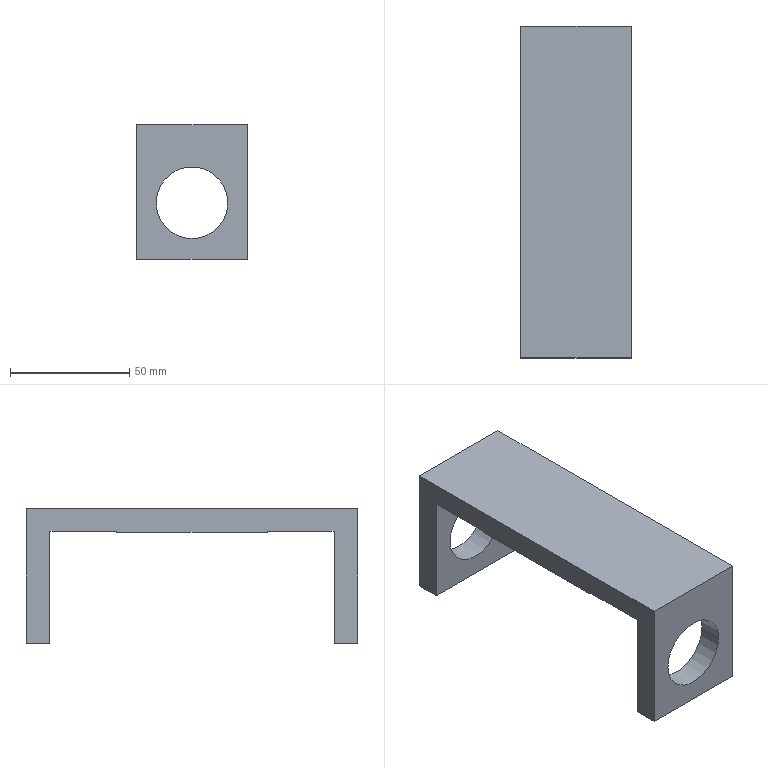Component | SolidWorks | HZ022-A001-D005-1 | 1 solid | 18 faces | box 46.5 x 139 x 56.5 mm | volume 92394 mm3 | plane 14 | cylinder 4 | commonest cylinder face diameters 30.05 x4 | material AL6061
build123d program:
from build123d import *

# Parameters (mm, degrees)
SKETCH1_2_W               = 139
SKETCH1_2_H               = 46.5
BOSS_EXTRUDE1_DEPTH       = 10
SKETCH2_W                 = 10
SKETCH2_H                 = 46.5
BOSS_EXTRUDE2_DEPTH       = 46.5
SKETCH3_R                 = 15.025
CUT_EXTRUDE1_DEPTH        = 152.835
SKETCH1_W                 = 28
SKETCH1_H                 = 60
CYLINDERCOVERRELIEF_DEPTH = 0.5


with BuildPart() as part:
    # Sketch1_2 → Boss-Extrude1 (new body)
    with BuildSketch(Plane(origin=(0, 0, 0), x_dir=(1, 0, 0), z_dir=(0, 1, 0))):
        Rectangle(SKETCH1_2_W, SKETCH1_2_H)
    extrude(amount=BOSS_EXTRUDE1_DEPTH)

    # Sketch2 → Boss-Extrude2 (add)
    with BuildSketch(Plane(origin=(0, 10, 0), x_dir=(1, 0, 0), z_dir=(0, 1, 0))):
        with Locations((-64.5, 0)):
            Rectangle(SKETCH2_W, SKETCH2_H)
        with Locations((64.5, 0)):
            Rectangle(SKETCH2_W, SKETCH2_H)
    extrude(amount=BOSS_EXTRUDE2_DEPTH)

    # Sketch3 → Cut-Extrude1 (cut, through all)
    with BuildSketch(Plane(origin=(69.5, 0, 0), x_dir=(0, 0, -1), z_dir=(1, 0, 0))):
        with Locations((0, 32.75)):
            Circle(SKETCH3_R)
    extrude(amount=-CUT_EXTRUDE1_DEPTH, mode=Mode.SUBTRACT)

    # Sketch1 → CylinderCoverRelief (cut)
    with BuildSketch(Plane(origin=(0, 10, 0), x_dir=(1, 0, 0), z_dir=(0, 1, 0))):
        with Locations((45.5, 0)):
            Rectangle(SKETCH1_W, SKETCH1_H)
        with Locations((-45.5, 0)):
            Rectangle(SKETCH1_W, SKETCH1_H)
    extrude(amount=-CYLINDERCOVERRELIEF_DEPTH, mode=Mode.SUBTRACT)


solid = part.part

# Placed as in the assembly
solid = solid.moved(Location((-12.865, -82.102, 400), (-90, 90, 0)))
STEP:
#1=COLOUR_RGB('',0.7922,0.8196,0.9333);
#2=FILL_AREA_STYLE_COLOUR('',#1);
#3=FILL_AREA_STYLE('',(#2));
#4=SURFACE_STYLE_FILL_AREA(#3);
#5=SURFACE_SIDE_STYLE('',(#4));
#6=SURFACE_STYLE_USAGE(.BOTH.,#5);
#7=PRESENTATION_STYLE_ASSIGNMENT((#6));
#8=CARTESIAN_POINT('',(0.08504,-0.4962,14.459));
#9=VERTEX_POINT('',#8);
#10=CARTESIAN_POINT('',(-1.098,-0.4962,14.459));
#11=VERTEX_POINT('',#10);
#12=CARTESIAN_POINT('',(-0.5065,-0.4962,14.459));
#13=DIRECTION('',(0.,-1.,0.));
#14=DIRECTION('',(-1.,0.,0.));
#15=AXIS2_PLACEMENT_3D('',#12,#13,#14);
#16=CIRCLE('',#15,0.5915);
#17=EDGE_CURVE('',#9,#11,#16,.T.);
#18=ORIENTED_EDGE('',*,*,#17,.F.);
#19=CARTESIAN_POINT('',(0.08504,-0.8899,14.459));
#20=VERTEX_POINT('',#19);
#21=CARTESIAN_POINT('',(0.08504,-0.4962,14.459));
#22=DIRECTION('',(0.,-1.,0.));
#23=VECTOR('',#22,39.37);
#24=LINE('',#21,#23);
#25=EDGE_CURVE('',#9,#20,#24,.T.);
#26=ORIENTED_EDGE('',*,*,#25,.T.);
#27=CARTESIAN_POINT('',(-1.098,-0.8899,14.459));
#28=VERTEX_POINT('',#27);
#29=CARTESIAN_POINT('',(-0.5065,-0.8899,14.459));
#30=DIRECTION('',(-0.,1.,-0.));
#31=DIRECTION('',(1.,0.,0.));
#32=AXIS2_PLACEMENT_3D('',#29,#30,#31);
#33=CIRCLE('',#32,0.5915);
#34=EDGE_CURVE('',#28,#20,#33,.T.);
#35=ORIENTED_EDGE('',*,*,#34,.F.);
#36=CARTESIAN_POINT('',(-1.098,-0.4962,14.459));
#37=DIRECTION('',(0.,-1.,0.));
#38=VECTOR('',#37,39.37);
#39=LINE('',#36,#38);
#40=EDGE_CURVE('',#11,#28,#39,.T.);
#41=ORIENTED_EDGE('',*,*,#40,.F.);
#42=EDGE_LOOP('',(#18,#26,#35,#41));
#43=FACE_OUTER_BOUND('',#42,.T.);
#44=CARTESIAN_POINT('',(-0.5065,-0.4962,14.459));
#45=DIRECTION('',(0.,-1.,0.));
#46=DIRECTION('',(-1.,0.,0.));
#47=AXIS2_PLACEMENT_3D('',#44,#45,#46);
#48=CYLINDRICAL_SURFACE('',#47,0.5915);
#49=ADVANCED_FACE('',(#43),#48,.F.);
#50=CARTESIAN_POINT('',(0.08504,-5.575,14.459));
#51=VERTEX_POINT('',#50);
#52=CARTESIAN_POINT('',(-1.098,-5.575,14.459));
#53=VERTEX_POINT('',#52);
#54=CARTESIAN_POINT('',(-0.5065,-5.575,14.459));
#55=DIRECTION('',(-0.,-1.,-0.));
#56=DIRECTION('',(-1.,0.,0.));
#57=AXIS2_PLACEMENT_3D('',#54,#55,#56);
#58=CIRCLE('',#57,0.5915);
#59=EDGE_CURVE('',#51,#53,#58,.T.);
#60=ORIENTED_EDGE('',*,*,#59,.F.);
#61=CARTESIAN_POINT('',(0.08504,-5.969,14.459));
#62=VERTEX_POINT('',#61);
#63=CARTESIAN_POINT('',(0.08504,-0.4962,14.459));
#64=DIRECTION('',(0.,-1.,0.));
#65=VECTOR('',#64,39.37);
#66=LINE('',#63,#65);
#67=EDGE_CURVE('',#51,#62,#66,.T.);
#68=ORIENTED_EDGE('',*,*,#67,.T.);
#69=CARTESIAN_POINT('',(-1.098,-5.969,14.459));
#70=VERTEX_POINT('',#69);
#71=CARTESIAN_POINT('',(-0.5065,-5.969,14.459));
#72=DIRECTION('',(0.,-1.,0.));
#73=DIRECTION('',(-1.,0.,0.));
#74=AXIS2_PLACEMENT_3D('',#71,#72,#73);
#75=CIRCLE('',#74,0.5915);
#76=EDGE_CURVE('',#62,#70,#75,.T.);
#77=ORIENTED_EDGE('',*,*,#76,.T.);
#78=CARTESIAN_POINT('',(-1.098,-0.4962,14.459));
#79=DIRECTION('',(0.,-1.,0.));
#80=VECTOR('',#79,39.37);
#81=LINE('',#78,#80);
#82=EDGE_CURVE('',#53,#70,#81,.T.);
#83=ORIENTED_EDGE('',*,*,#82,.F.);
#84=EDGE_LOOP('',(#60,#68,#77,#83));
#85=FACE_OUTER_BOUND('',#84,.T.);
#86=CARTESIAN_POINT('',(-0.5065,-0.4962,14.459));
#87=DIRECTION('',(0.,-1.,0.));
#88=DIRECTION('',(-1.,0.,0.));
#89=AXIS2_PLACEMENT_3D('',#86,#87,#88);
#90=CYLINDRICAL_SURFACE('',#89,0.5915);
#91=ADVANCED_FACE('',(#85),#90,.F.);
#92=CARTESIAN_POINT('',(-1.422,-4.473,15.354));
#93=VERTEX_POINT('',#92);
#94=CARTESIAN_POINT('',(0.4089,-4.473,15.354));
#95=VERTEX_POINT('',#94);
#96=CARTESIAN_POINT('',(0.6746,-4.473,15.354));
#97=DIRECTION('',(1.,-0.,0.));
#98=VECTOR('',#97,39.37);
#99=LINE('',#96,#98);
#100=EDGE_CURVE('',#93,#95,#99,.T.);
#101=ORIENTED_EDGE('',*,*,#100,.F.);
#102=CARTESIAN_POINT('',(-1.422,-1.992,15.354));
#103=VERTEX_POINT('',#102);
#104=CARTESIAN_POINT('',(-1.422,-0.4962,15.354));
#105=DIRECTION('',(-0.,1.,-0.));
#106=VECTOR('',#105,39.37);
#107=LINE('',#104,#106);
#108=EDGE_CURVE('',#93,#103,#107,.T.);
#109=ORIENTED_EDGE('',*,*,#108,.T.);
#110=CARTESIAN_POINT('',(0.4089,-1.992,15.354));
#111=VERTEX_POINT('',#110);
#112=CARTESIAN_POINT('',(-1.688,-1.992,15.354));
#113=DIRECTION('',(-1.,0.,-0.));
#114=VECTOR('',#113,39.37);
#115=LINE('',#112,#114);
#116=EDGE_CURVE('',#111,#103,#115,.T.);
#117=ORIENTED_EDGE('',*,*,#116,.F.);
#118=CARTESIAN_POINT('',(0.4089,-0.4962,15.354));
#119=DIRECTION('',(0.,-1.,0.));
#120=VECTOR('',#119,39.37);
#121=LINE('',#118,#120);
#122=EDGE_CURVE('',#111,#95,#121,.T.);
#123=ORIENTED_EDGE('',*,*,#122,.T.);
#124=EDGE_LOOP('',(#101,#109,#117,#123));
#125=FACE_OUTER_BOUND('',#124,.T.);
#126=CARTESIAN_POINT('',(-0.5065,-3.232,15.354));
#127=DIRECTION('',(0.,0.,-1.));
#128=DIRECTION('',(1.,-0.,0.));
#129=AXIS2_PLACEMENT_3D('',#126,#127,#128);
#130=PLANE('',#129);
#131=ADVANCED_FACE('',(#125),#130,.T.);
#132=CARTESIAN_POINT('',(-0.5065,-5.969,14.459));
#133=DIRECTION('',(0.,-1.,0.));
#134=DIRECTION('',(-1.,0.,0.));
#135=AXIS2_PLACEMENT_3D('',#132,#133,#134);
#136=CIRCLE('',#135,0.5915);
#137=EDGE_CURVE('',#70,#62,#136,.T.);
#138=ORIENTED_EDGE('',*,*,#137,.F.);
#139=ORIENTED_EDGE('',*,*,#76,.F.);
#140=EDGE_LOOP('',(#138,#139));
#141=FACE_BOUND('',#140,.T.);
#142=CARTESIAN_POINT('',(0.4089,-5.969,15.748));
#143=VERTEX_POINT('',#142);
#144=CARTESIAN_POINT('',(-1.422,-5.969,15.748));
#145=VERTEX_POINT('',#144);
#146=CARTESIAN_POINT('',(-1.422,-5.969,15.748));
#147=DIRECTION('',(-1.,0.,-0.));
#148=VECTOR('',#147,39.37);
#149=LINE('',#146,#148);
#150=EDGE_CURVE('',#143,#145,#149,.T.);
#151=ORIENTED_EDGE('',*,*,#150,.T.);
#152=CARTESIAN_POINT('',(-1.422,-5.969,13.524));
#153=VERTEX_POINT('',#152);
#154=CARTESIAN_POINT('',(-1.422,-5.969,15.354));
#155=DIRECTION('',(-0.,-0.,1.));
#156=VECTOR('',#155,39.37);
#157=LINE('',#154,#156);
#158=EDGE_CURVE('',#153,#145,#157,.T.);
#159=ORIENTED_EDGE('',*,*,#158,.F.);
#160=CARTESIAN_POINT('',(0.4089,-5.969,13.524));
#161=VERTEX_POINT('',#160);
#162=CARTESIAN_POINT('',(0.4089,-5.969,13.524));
#163=DIRECTION('',(-1.,0.,-0.));
#164=VECTOR('',#163,39.37);
#165=LINE('',#162,#164);
#166=EDGE_CURVE('',#161,#153,#165,.T.);
#167=ORIENTED_EDGE('',*,*,#166,.F.);
#168=CARTESIAN_POINT('',(0.4089,-5.969,15.354));
#169=DIRECTION('',(-0.,-0.,1.));
#170=VECTOR('',#169,39.37);
#171=LINE('',#168,#170);
#172=EDGE_CURVE('',#161,#143,#171,.T.);
#173=ORIENTED_EDGE('',*,*,#172,.T.);
#174=EDGE_LOOP('',(#151,#159,#167,#173));
#175=FACE_OUTER_BOUND('',#174,.T.);
#176=CARTESIAN_POINT('',(-1.422,-5.969,15.354));
#177=DIRECTION('',(0.,1.,-0.));
#178=DIRECTION('',(1.,-0.,0.));
#179=AXIS2_PLACEMENT_3D('',#176,#177,#178);
#180=PLANE('',#179);
#181=ADVANCED_FACE('',(#141,#175),#180,.F.);
#182=ORIENTED_EDGE('',*,*,#108,.F.);
#183=CARTESIAN_POINT('',(-1.422,-4.473,15.374));
#184=VERTEX_POINT('',#183);
#185=CARTESIAN_POINT('',(-1.422,-4.473,15.354));
#186=DIRECTION('',(-0.,-0.,1.));
#187=VECTOR('',#186,39.37);
#188=LINE('',#185,#187);
#189=EDGE_CURVE('',#93,#184,#188,.T.);
#190=ORIENTED_EDGE('',*,*,#189,.T.);
#191=CARTESIAN_POINT('',(-1.422,-5.575,15.374));
#192=VERTEX_POINT('',#191);
#193=CARTESIAN_POINT('',(-1.422,-0.4962,15.374));
#194=DIRECTION('',(0.,-1.,0.));
#195=VECTOR('',#194,39.37);
#196=LINE('',#193,#195);
#197=EDGE_CURVE('',#184,#192,#196,.T.);
#198=ORIENTED_EDGE('',*,*,#197,.T.);
#199=CARTESIAN_POINT('',(-1.422,-5.575,13.524));
#200=VERTEX_POINT('',#199);
#201=CARTESIAN_POINT('',(-1.422,-5.575,13.524));
#202=DIRECTION('',(-0.,-0.,1.));
#203=VECTOR('',#202,39.37);
#204=LINE('',#201,#203);
#205=EDGE_CURVE('',#200,#192,#204,.T.);
#206=ORIENTED_EDGE('',*,*,#205,.F.);
#207=CARTESIAN_POINT('',(-1.422,-5.575,13.524));
#208=DIRECTION('',(-0.,1.,-0.));
#209=VECTOR('',#208,39.37);
#210=LINE('',#207,#209);
#211=EDGE_CURVE('',#153,#200,#210,.T.);
#212=ORIENTED_EDGE('',*,*,#211,.F.);
#213=ORIENTED_EDGE('',*,*,#158,.T.);
#214=CARTESIAN_POINT('',(-1.422,-0.4962,15.748));
#215=VERTEX_POINT('',#214);
#216=CARTESIAN_POINT('',(-1.422,-0.4962,15.748));
#217=DIRECTION('',(-0.,1.,-0.));
#218=VECTOR('',#217,39.37);
#219=LINE('',#216,#218);
#220=EDGE_CURVE('',#145,#215,#219,.T.);
#221=ORIENTED_EDGE('',*,*,#220,.T.);
#222=CARTESIAN_POINT('',(-1.422,-0.4962,13.524));
#223=VERTEX_POINT('',#222);
#224=CARTESIAN_POINT('',(-1.422,-0.4962,15.354));
#225=DIRECTION('',(-0.,-0.,1.));
#226=VECTOR('',#225,39.37);
#227=LINE('',#224,#226);
#228=EDGE_CURVE('',#223,#215,#227,.T.);
#229=ORIENTED_EDGE('',*,*,#228,.F.);
#230=CARTESIAN_POINT('',(-1.422,-0.8899,13.524));
#231=VERTEX_POINT('',#230);
#232=CARTESIAN_POINT('',(-1.422,-0.8899,13.524));
#233=DIRECTION('',(-0.,1.,-0.));
#234=VECTOR('',#233,39.37);
#235=LINE('',#232,#234);
#236=EDGE_CURVE('',#231,#223,#235,.T.);
#237=ORIENTED_EDGE('',*,*,#236,.F.);
#238=CARTESIAN_POINT('',(-1.422,-0.8899,15.374));
#239=VERTEX_POINT('',#238);
#240=CARTESIAN_POINT('',(-1.422,-0.8899,13.524));
#241=DIRECTION('',(-0.,-0.,1.));
#242=VECTOR('',#241,39.37);
#243=LINE('',#240,#242);
#244=EDGE_CURVE('',#231,#239,#243,.T.);
#245=ORIENTED_EDGE('',*,*,#244,.T.);
#246=CARTESIAN_POINT('',(-1.422,-1.992,15.374));
#247=VERTEX_POINT('',#246);
#248=CARTESIAN_POINT('',(-1.422,-0.4962,15.374));
#249=DIRECTION('',(0.,-1.,0.));
#250=VECTOR('',#249,39.37);
#251=LINE('',#248,#250);
#252=EDGE_CURVE('',#239,#247,#251,.T.);
#253=ORIENTED_EDGE('',*,*,#252,.T.);
#254=CARTESIAN_POINT('',(-1.422,-1.992,15.354));
#255=DIRECTION('',(0.,0.,-1.));
#256=VECTOR('',#255,39.37);
#257=LINE('',#254,#256);
#258=EDGE_CURVE('',#247,#103,#257,.T.);
#259=ORIENTED_EDGE('',*,*,#258,.T.);
#260=EDGE_LOOP('',(#182,#190,#198,#206,#212,#213,#221,#229,#237,#245,#253,#259));
#261=FACE_OUTER_BOUND('',#260,.T.);
#262=CARTESIAN_POINT('',(-1.422,-0.4962,15.354));
#263=DIRECTION('',(1.,0.,0.));
#264=DIRECTION('',(0.,-1.,0.));
#265=AXIS2_PLACEMENT_3D('',#262,#263,#264);
#266=PLANE('',#265);
#267=ADVANCED_FACE('',(#261),#266,.F.);
#268=CARTESIAN_POINT('',(-0.5065,-0.4962,14.459));
#269=DIRECTION('',(0.,-1.,0.));
#270=DIRECTION('',(-1.,0.,0.));
#271=AXIS2_PLACEMENT_3D('',#268,#269,#270);
#272=CIRCLE('',#271,0.5915);
#273=EDGE_CURVE('',#11,#9,#272,.T.);
#274=ORIENTED_EDGE('',*,*,#273,.T.);
#275=ORIENTED_EDGE('',*,*,#17,.T.);
#276=EDGE_LOOP('',(#274,#275));
#277=FACE_BOUND('',#276,.T.);
#278=CARTESIAN_POINT('',(0.4089,-0.4962,15.748));
#279=VERTEX_POINT('',#278);
#280=CARTESIAN_POINT('',(-1.422,-0.4962,15.748));
#281=DIRECTION('',(1.,-0.,0.));
#282=VECTOR('',#281,39.37);
#283=LINE('',#280,#282);
#284=EDGE_CURVE('',#215,#279,#283,.T.);
#285=ORIENTED_EDGE('',*,*,#284,.T.);
#286=CARTESIAN_POINT('',(0.4089,-0.4962,13.524));
#287=VERTEX_POINT('',#286);
#288=CARTESIAN_POINT('',(0.4089,-0.4962,15.354));
#289=DIRECTION('',(-0.,-0.,1.));
#290=VECTOR('',#289,39.37);
#291=LINE('',#288,#290);
#292=EDGE_CURVE('',#287,#279,#291,.T.);
#293=ORIENTED_EDGE('',*,*,#292,.F.);
#294=CARTESIAN_POINT('',(0.4089,-0.4962,13.524));
#295=DIRECTION('',(1.,-0.,0.));
#296=VECTOR('',#295,39.37);
#297=LINE('',#294,#296);
#298=EDGE_CURVE('',#223,#287,#297,.T.);
#299=ORIENTED_EDGE('',*,*,#298,.F.);
#300=ORIENTED_EDGE('',*,*,#228,.T.);
#301=EDGE_LOOP('',(#285,#293,#299,#300));
#302=FACE_OUTER_BOUND('',#301,.T.);
#303=CARTESIAN_POINT('',(-1.422,-0.4962,15.354));
#304=DIRECTION('',(-0.,-1.,0.));
#305=DIRECTION('',(-1.,0.,-0.));
#306=AXIS2_PLACEMENT_3D('',#303,#304,#305);
#307=PLANE('',#306);
#308=ADVANCED_FACE('',(#277,#302),#307,.F.);
#309=CARTESIAN_POINT('',(0.4089,-5.575,15.374));
#310=VERTEX_POINT('',#309);
#311=CARTESIAN_POINT('',(0.4089,-4.473,15.374));
#312=VERTEX_POINT('',#311);
#313=CARTESIAN_POINT('',(0.4089,-0.4962,15.374));
#314=DIRECTION('',(-0.,1.,-0.));
#315=VECTOR('',#314,39.37);
#316=LINE('',#313,#315);
#317=EDGE_CURVE('',#310,#312,#316,.T.);
#318=ORIENTED_EDGE('',*,*,#317,.T.);
#319=CARTESIAN_POINT('',(0.4089,-4.473,15.354));
#320=DIRECTION('',(0.,0.,-1.));
#321=VECTOR('',#320,39.37);
#322=LINE('',#319,#321);
#323=EDGE_CURVE('',#312,#95,#322,.T.);
#324=ORIENTED_EDGE('',*,*,#323,.T.);
#325=ORIENTED_EDGE('',*,*,#122,.F.);
#326=CARTESIAN_POINT('',(0.4089,-1.992,15.374));
#327=VERTEX_POINT('',#326);
#328=CARTESIAN_POINT('',(0.4089,-1.992,15.354));
#329=DIRECTION('',(-0.,-0.,1.));
#330=VECTOR('',#329,39.37);
#331=LINE('',#328,#330);
#332=EDGE_CURVE('',#111,#327,#331,.T.);
#333=ORIENTED_EDGE('',*,*,#332,.T.);
#334=CARTESIAN_POINT('',(0.4089,-0.8899,15.374));
#335=VERTEX_POINT('',#334);
#336=CARTESIAN_POINT('',(0.4089,-0.4962,15.374));
#337=DIRECTION('',(-0.,1.,-0.));
#338=VECTOR('',#337,39.37);
#339=LINE('',#336,#338);
#340=EDGE_CURVE('',#327,#335,#339,.T.);
#341=ORIENTED_EDGE('',*,*,#340,.T.);
#342=CARTESIAN_POINT('',(0.4089,-0.8899,13.524));
#343=VERTEX_POINT('',#342);
#344=CARTESIAN_POINT('',(0.4089,-0.8899,13.524));
#345=DIRECTION('',(-0.,-0.,1.));
#346=VECTOR('',#345,39.37);
#347=LINE('',#344,#346);
#348=EDGE_CURVE('',#343,#335,#347,.T.);
#349=ORIENTED_EDGE('',*,*,#348,.F.);
#350=CARTESIAN_POINT('',(0.4089,-0.8899,13.524));
#351=DIRECTION('',(0.,-1.,0.));
#352=VECTOR('',#351,39.37);
#353=LINE('',#350,#352);
#354=EDGE_CURVE('',#287,#343,#353,.T.);
#355=ORIENTED_EDGE('',*,*,#354,.F.);
#356=ORIENTED_EDGE('',*,*,#292,.T.);
#357=CARTESIAN_POINT('',(0.4089,-0.4962,15.748));
#358=DIRECTION('',(0.,-1.,0.));
#359=VECTOR('',#358,39.37);
#360=LINE('',#357,#359);
#361=EDGE_CURVE('',#279,#143,#360,.T.);
#362=ORIENTED_EDGE('',*,*,#361,.T.);
#363=ORIENTED_EDGE('',*,*,#172,.F.);
#364=CARTESIAN_POINT('',(0.4089,-5.575,13.524));
#365=VERTEX_POINT('',#364);
#366=CARTESIAN_POINT('',(0.4089,-5.575,13.524));
#367=DIRECTION('',(-0.,-1.,-0.));
#368=VECTOR('',#367,39.37);
#369=LINE('',#366,#368);
#370=EDGE_CURVE('',#365,#161,#369,.T.);
#371=ORIENTED_EDGE('',*,*,#370,.F.);
#372=CARTESIAN_POINT('',(0.4089,-5.575,13.524));
#373=DIRECTION('',(-0.,-0.,1.));
#374=VECTOR('',#373,39.37);
#375=LINE('',#372,#374);
#376=EDGE_CURVE('',#365,#310,#375,.T.);
#377=ORIENTED_EDGE('',*,*,#376,.T.);
#378=EDGE_LOOP('',(#318,#324,#325,#333,#341,#349,#355,#356,#362,#363,#371,#377));
#379=FACE_OUTER_BOUND('',#378,.T.);
#380=CARTESIAN_POINT('',(0.4089,-0.4962,15.354));
#381=DIRECTION('',(-1.,-0.,-0.));
#382=DIRECTION('',(-0.,1.,-0.));
#383=AXIS2_PLACEMENT_3D('',#380,#381,#382);
#384=PLANE('',#383);
#385=ADVANCED_FACE('',(#379),#384,.F.);
#386=ORIENTED_EDGE('',*,*,#150,.F.);
#387=ORIENTED_EDGE('',*,*,#361,.F.);
#388=ORIENTED_EDGE('',*,*,#284,.F.);
#389=ORIENTED_EDGE('',*,*,#220,.F.);
#390=EDGE_LOOP('',(#386,#387,#388,#389));
#391=FACE_OUTER_BOUND('',#390,.T.);
#392=CARTESIAN_POINT('',(-0.5065,-3.232,15.748));
#393=DIRECTION('',(0.,0.,-1.));
#394=DIRECTION('',(1.,-0.,0.));
#395=AXIS2_PLACEMENT_3D('',#392,#393,#394);
#396=PLANE('',#395);
#397=ADVANCED_FACE('',(#391),#396,.F.);
#398=ORIENTED_EDGE('',*,*,#34,.T.);
#399=CARTESIAN_POINT('',(-0.5065,-0.8899,14.459));
#400=DIRECTION('',(-0.,1.,-0.));
#401=DIRECTION('',(1.,0.,0.));
#402=AXIS2_PLACEMENT_3D('',#399,#400,#401);
#403=CIRCLE('',#402,0.5915);
#404=EDGE_CURVE('',#20,#28,#403,.T.);
#405=ORIENTED_EDGE('',*,*,#404,.T.);
#406=EDGE_LOOP('',(#398,#405));
#407=FACE_BOUND('',#406,.T.);
#408=ORIENTED_EDGE('',*,*,#348,.T.);
#409=CARTESIAN_POINT('',(0.6746,-0.8899,15.374));
#410=DIRECTION('',(1.,-0.,0.));
#411=VECTOR('',#410,39.37);
#412=LINE('',#409,#411);
#413=EDGE_CURVE('',#239,#335,#412,.T.);
#414=ORIENTED_EDGE('',*,*,#413,.F.);
#415=ORIENTED_EDGE('',*,*,#244,.F.);
#416=CARTESIAN_POINT('',(0.4089,-0.8899,13.524));
#417=DIRECTION('',(-1.,0.,-0.));
#418=VECTOR('',#417,39.37);
#419=LINE('',#416,#418);
#420=EDGE_CURVE('',#343,#231,#419,.T.);
#421=ORIENTED_EDGE('',*,*,#420,.F.);
#422=EDGE_LOOP('',(#408,#414,#415,#421));
#423=FACE_OUTER_BOUND('',#422,.T.);
#424=CARTESIAN_POINT('',(0.4089,-0.8899,13.524));
#425=DIRECTION('',(0.,1.,-0.));
#426=DIRECTION('',(1.,-0.,0.));
#427=AXIS2_PLACEMENT_3D('',#424,#425,#426);
#428=PLANE('',#427);
#429=ADVANCED_FACE('',(#407,#423),#428,.F.);
#430=ORIENTED_EDGE('',*,*,#298,.T.);
#431=ORIENTED_EDGE('',*,*,#354,.T.);
#432=ORIENTED_EDGE('',*,*,#420,.T.);
#433=ORIENTED_EDGE('',*,*,#236,.T.);
#434=EDGE_LOOP('',(#430,#431,#432,#433));
#435=FACE_OUTER_BOUND('',#434,.T.);
#436=CARTESIAN_POINT('',(-0.5065,-3.232,13.524));
#437=DIRECTION('',(0.,0.,-1.));
#438=DIRECTION('',(1.,-0.,0.));
#439=AXIS2_PLACEMENT_3D('',#436,#437,#438);
#440=PLANE('',#439);
#441=ADVANCED_FACE('',(#435),#440,.T.);
#442=CARTESIAN_POINT('',(-0.5065,-5.575,14.459));
#443=DIRECTION('',(-0.,-1.,-0.));
#444=DIRECTION('',(-1.,0.,0.));
#445=AXIS2_PLACEMENT_3D('',#442,#443,#444);
#446=CIRCLE('',#445,0.5915);
#447=EDGE_CURVE('',#53,#51,#446,.T.);
#448=ORIENTED_EDGE('',*,*,#447,.T.);
#449=ORIENTED_EDGE('',*,*,#59,.T.);
#450=EDGE_LOOP('',(#448,#449));
#451=FACE_BOUND('',#450,.T.);
#452=ORIENTED_EDGE('',*,*,#205,.T.);
#453=CARTESIAN_POINT('',(-1.688,-5.575,15.374));
#454=DIRECTION('',(-1.,0.,-0.));
#455=VECTOR('',#454,39.37);
#456=LINE('',#453,#455);
#457=EDGE_CURVE('',#310,#192,#456,.T.);
#458=ORIENTED_EDGE('',*,*,#457,.F.);
#459=ORIENTED_EDGE('',*,*,#376,.F.);
#460=CARTESIAN_POINT('',(0.4089,-5.575,13.524));
#461=DIRECTION('',(1.,-0.,0.));
#462=VECTOR('',#461,39.37);
#463=LINE('',#460,#462);
#464=EDGE_CURVE('',#200,#365,#463,.T.);
#465=ORIENTED_EDGE('',*,*,#464,.F.);
#466=EDGE_LOOP('',(#452,#458,#459,#465));
#467=FACE_OUTER_BOUND('',#466,.T.);
#468=CARTESIAN_POINT('',(0.4089,-5.575,13.524));
#469=DIRECTION('',(-0.,-1.,-0.));
#470=DIRECTION('',(-1.,0.,-0.));
#471=AXIS2_PLACEMENT_3D('',#468,#469,#470);
#472=PLANE('',#471);
#473=ADVANCED_FACE('',(#451,#467),#472,.F.);
#474=ORIENTED_EDGE('',*,*,#464,.T.);
#475=ORIENTED_EDGE('',*,*,#370,.T.);
#476=ORIENTED_EDGE('',*,*,#166,.T.);
#477=ORIENTED_EDGE('',*,*,#211,.T.);
#478=EDGE_LOOP('',(#474,#475,#476,#477));
#479=FACE_OUTER_BOUND('',#478,.T.);
#480=CARTESIAN_POINT('',(-0.5065,-3.232,13.524));
#481=DIRECTION('',(-0.,-0.,1.));
#482=DIRECTION('',(-1.,0.,-0.));
#483=AXIS2_PLACEMENT_3D('',#480,#481,#482);
#484=PLANE('',#483);
#485=ADVANCED_FACE('',(#479),#484,.F.);
#486=ORIENTED_EDGE('',*,*,#67,.F.);
#487=ORIENTED_EDGE('',*,*,#447,.F.);
#488=ORIENTED_EDGE('',*,*,#82,.T.);
#489=ORIENTED_EDGE('',*,*,#137,.T.);
#490=EDGE_LOOP('',(#486,#487,#488,#489));
#491=FACE_OUTER_BOUND('',#490,.T.);
#492=CARTESIAN_POINT('',(-0.5065,-0.4962,14.459));
#493=DIRECTION('',(0.,-1.,0.));
#494=DIRECTION('',(-1.,0.,0.));
#495=AXIS2_PLACEMENT_3D('',#492,#493,#494);
#496=CYLINDRICAL_SURFACE('',#495,0.5915);
#497=ADVANCED_FACE('',(#491),#496,.F.);
#498=ORIENTED_EDGE('',*,*,#25,.F.);
#499=ORIENTED_EDGE('',*,*,#273,.F.);
#500=ORIENTED_EDGE('',*,*,#40,.T.);
#501=ORIENTED_EDGE('',*,*,#404,.F.);
#502=EDGE_LOOP('',(#498,#499,#500,#501));
#503=FACE_OUTER_BOUND('',#502,.T.);
#504=CARTESIAN_POINT('',(-0.5065,-0.4962,14.459));
#505=DIRECTION('',(0.,-1.,0.));
#506=DIRECTION('',(-1.,0.,0.));
#507=AXIS2_PLACEMENT_3D('',#504,#505,#506);
#508=CYLINDRICAL_SURFACE('',#507,0.5915);
#509=ADVANCED_FACE('',(#503),#508,.F.);
#510=CARTESIAN_POINT('',(-1.688,-1.992,15.374));
#511=DIRECTION('',(-1.,0.,-0.));
#512=VECTOR('',#511,39.37);
#513=LINE('',#510,#512);
#514=EDGE_CURVE('',#327,#247,#513,.T.);
#515=ORIENTED_EDGE('',*,*,#514,.F.);
#516=ORIENTED_EDGE('',*,*,#332,.F.);
#517=ORIENTED_EDGE('',*,*,#116,.T.);
#518=ORIENTED_EDGE('',*,*,#258,.F.);
#519=EDGE_LOOP('',(#515,#516,#517,#518));
#520=FACE_OUTER_BOUND('',#519,.T.);
#521=CARTESIAN_POINT('',(-1.688,-1.992,15.374));
#522=DIRECTION('',(-0.,-1.,0.));
#523=DIRECTION('',(-1.,0.,-0.));
#524=AXIS2_PLACEMENT_3D('',#521,#522,#523);
#525=PLANE('',#524);
#526=ADVANCED_FACE('',(#520),#525,.F.);
#527=ORIENTED_EDGE('',*,*,#413,.T.);
#528=ORIENTED_EDGE('',*,*,#340,.F.);
#529=ORIENTED_EDGE('',*,*,#514,.T.);
#530=ORIENTED_EDGE('',*,*,#252,.F.);
#531=EDGE_LOOP('',(#527,#528,#529,#530));
#532=FACE_OUTER_BOUND('',#531,.T.);
#533=CARTESIAN_POINT('',(-0.5065,-3.232,15.374));
#534=DIRECTION('',(-0.,-0.,1.));
#535=DIRECTION('',(-1.,0.,-0.));
#536=AXIS2_PLACEMENT_3D('',#533,#534,#535);
#537=PLANE('',#536);
#538=ADVANCED_FACE('',(#532),#537,.F.);
#539=ORIENTED_EDGE('',*,*,#100,.T.);
#540=ORIENTED_EDGE('',*,*,#323,.F.);
#541=CARTESIAN_POINT('',(0.6746,-4.473,15.374));
#542=DIRECTION('',(1.,-0.,0.));
#543=VECTOR('',#542,39.37);
#544=LINE('',#541,#543);
#545=EDGE_CURVE('',#184,#312,#544,.T.);
#546=ORIENTED_EDGE('',*,*,#545,.F.);
#547=ORIENTED_EDGE('',*,*,#189,.F.);
#548=EDGE_LOOP('',(#539,#540,#546,#547));
#549=FACE_OUTER_BOUND('',#548,.T.);
#550=CARTESIAN_POINT('',(0.6746,-4.473,15.374));
#551=DIRECTION('',(0.,1.,-0.));
#552=DIRECTION('',(1.,-0.,0.));
#553=AXIS2_PLACEMENT_3D('',#550,#551,#552);
#554=PLANE('',#553);
#555=ADVANCED_FACE('',(#549),#554,.F.);
#556=ORIENTED_EDGE('',*,*,#545,.T.);
#557=ORIENTED_EDGE('',*,*,#317,.F.);
#558=ORIENTED_EDGE('',*,*,#457,.T.);
#559=ORIENTED_EDGE('',*,*,#197,.F.);
#560=EDGE_LOOP('',(#556,#557,#558,#559));
#561=FACE_OUTER_BOUND('',#560,.T.);
#562=CARTESIAN_POINT('',(-0.5065,-3.232,15.374));
#563=DIRECTION('',(-0.,-0.,1.));
#564=DIRECTION('',(-1.,0.,-0.));
#565=AXIS2_PLACEMENT_3D('',#562,#563,#564);
#566=PLANE('',#565);
#567=ADVANCED_FACE('',(#561),#566,.F.);
#568=CLOSED_SHELL('',(#49,#91,#131,#181,#267,#308,#385,#397,#429,#441,#473,#485,#497,#509,#526,#538,#555,#567));
#569=MANIFOLD_SOLID_BREP('',#568);
#570=STYLED_ITEM('',(#7),#569);
#571=PRESENTATION_LAYER_ASSIGNMENT('','',(#570));
#572=CARTESIAN_POINT('',(0.,0.,0.));
#573=DIRECTION('',(0.,0.,1.));
#574=DIRECTION('',(1.,0.,0.));
#575=AXIS2_PLACEMENT_3D('',#572,#573,#574);
#576=(LENGTH_UNIT()NAMED_UNIT(*)SI_UNIT($,.METRE.));
#577=LENGTH_MEASURE_WITH_UNIT(LENGTH_MEASURE(0.0254),#576);
#578=DIMENSIONAL_EXPONENTS(1.,0.,0.,0.,0.,0.,0.);
#579=(CONVERSION_BASED_UNIT('',#577)LENGTH_UNIT()NAMED_UNIT(#578));
#580=UNCERTAINTY_MEASURE_WITH_UNIT(LENGTH_MEASURE(0.00001),#579,'','');
#581=(NAMED_UNIT(*)PLANE_ANGLE_UNIT()SI_UNIT($,.RADIAN.));
#582=(NAMED_UNIT(*)SI_UNIT($,.STERADIAN.)SOLID_ANGLE_UNIT());
#583=(GEOMETRIC_REPRESENTATION_CONTEXT(3)GLOBAL_UNCERTAINTY_ASSIGNED_CONTEXT((#580))GLOBAL_UNIT_ASSIGNED_CONTEXT((#579,#581,#582))REPRESENTATION_CONTEXT('',''));
#584=ADVANCED_BREP_SHAPE_REPRESENTATION('',(#569,#575),#583);
#585=(LENGTH_UNIT()NAMED_UNIT(*)SI_UNIT($,.METRE.));
#586=LENGTH_MEASURE_WITH_UNIT(LENGTH_MEASURE(0.0254),#585);
#587=DIMENSIONAL_EXPONENTS(1.,0.,0.,0.,0.,0.,0.);
#588=(CONVERSION_BASED_UNIT('',#586)LENGTH_UNIT()NAMED_UNIT(#587));
#589=UNCERTAINTY_MEASURE_WITH_UNIT(LENGTH_MEASURE(0.00001),#588,'','');
#590=(NAMED_UNIT(*)PLANE_ANGLE_UNIT()SI_UNIT($,.RADIAN.));
#591=(NAMED_UNIT(*)SI_UNIT($,.STERADIAN.)SOLID_ANGLE_UNIT());
#592=(GEOMETRIC_REPRESENTATION_CONTEXT(3)GLOBAL_UNCERTAINTY_ASSIGNED_CONTEXT((#589))GLOBAL_UNIT_ASSIGNED_CONTEXT((#588,#590,#591))REPRESENTATION_CONTEXT('',''));
#593=MECHANICAL_DESIGN_GEOMETRIC_PRESENTATION_REPRESENTATION('',(#570),#592);